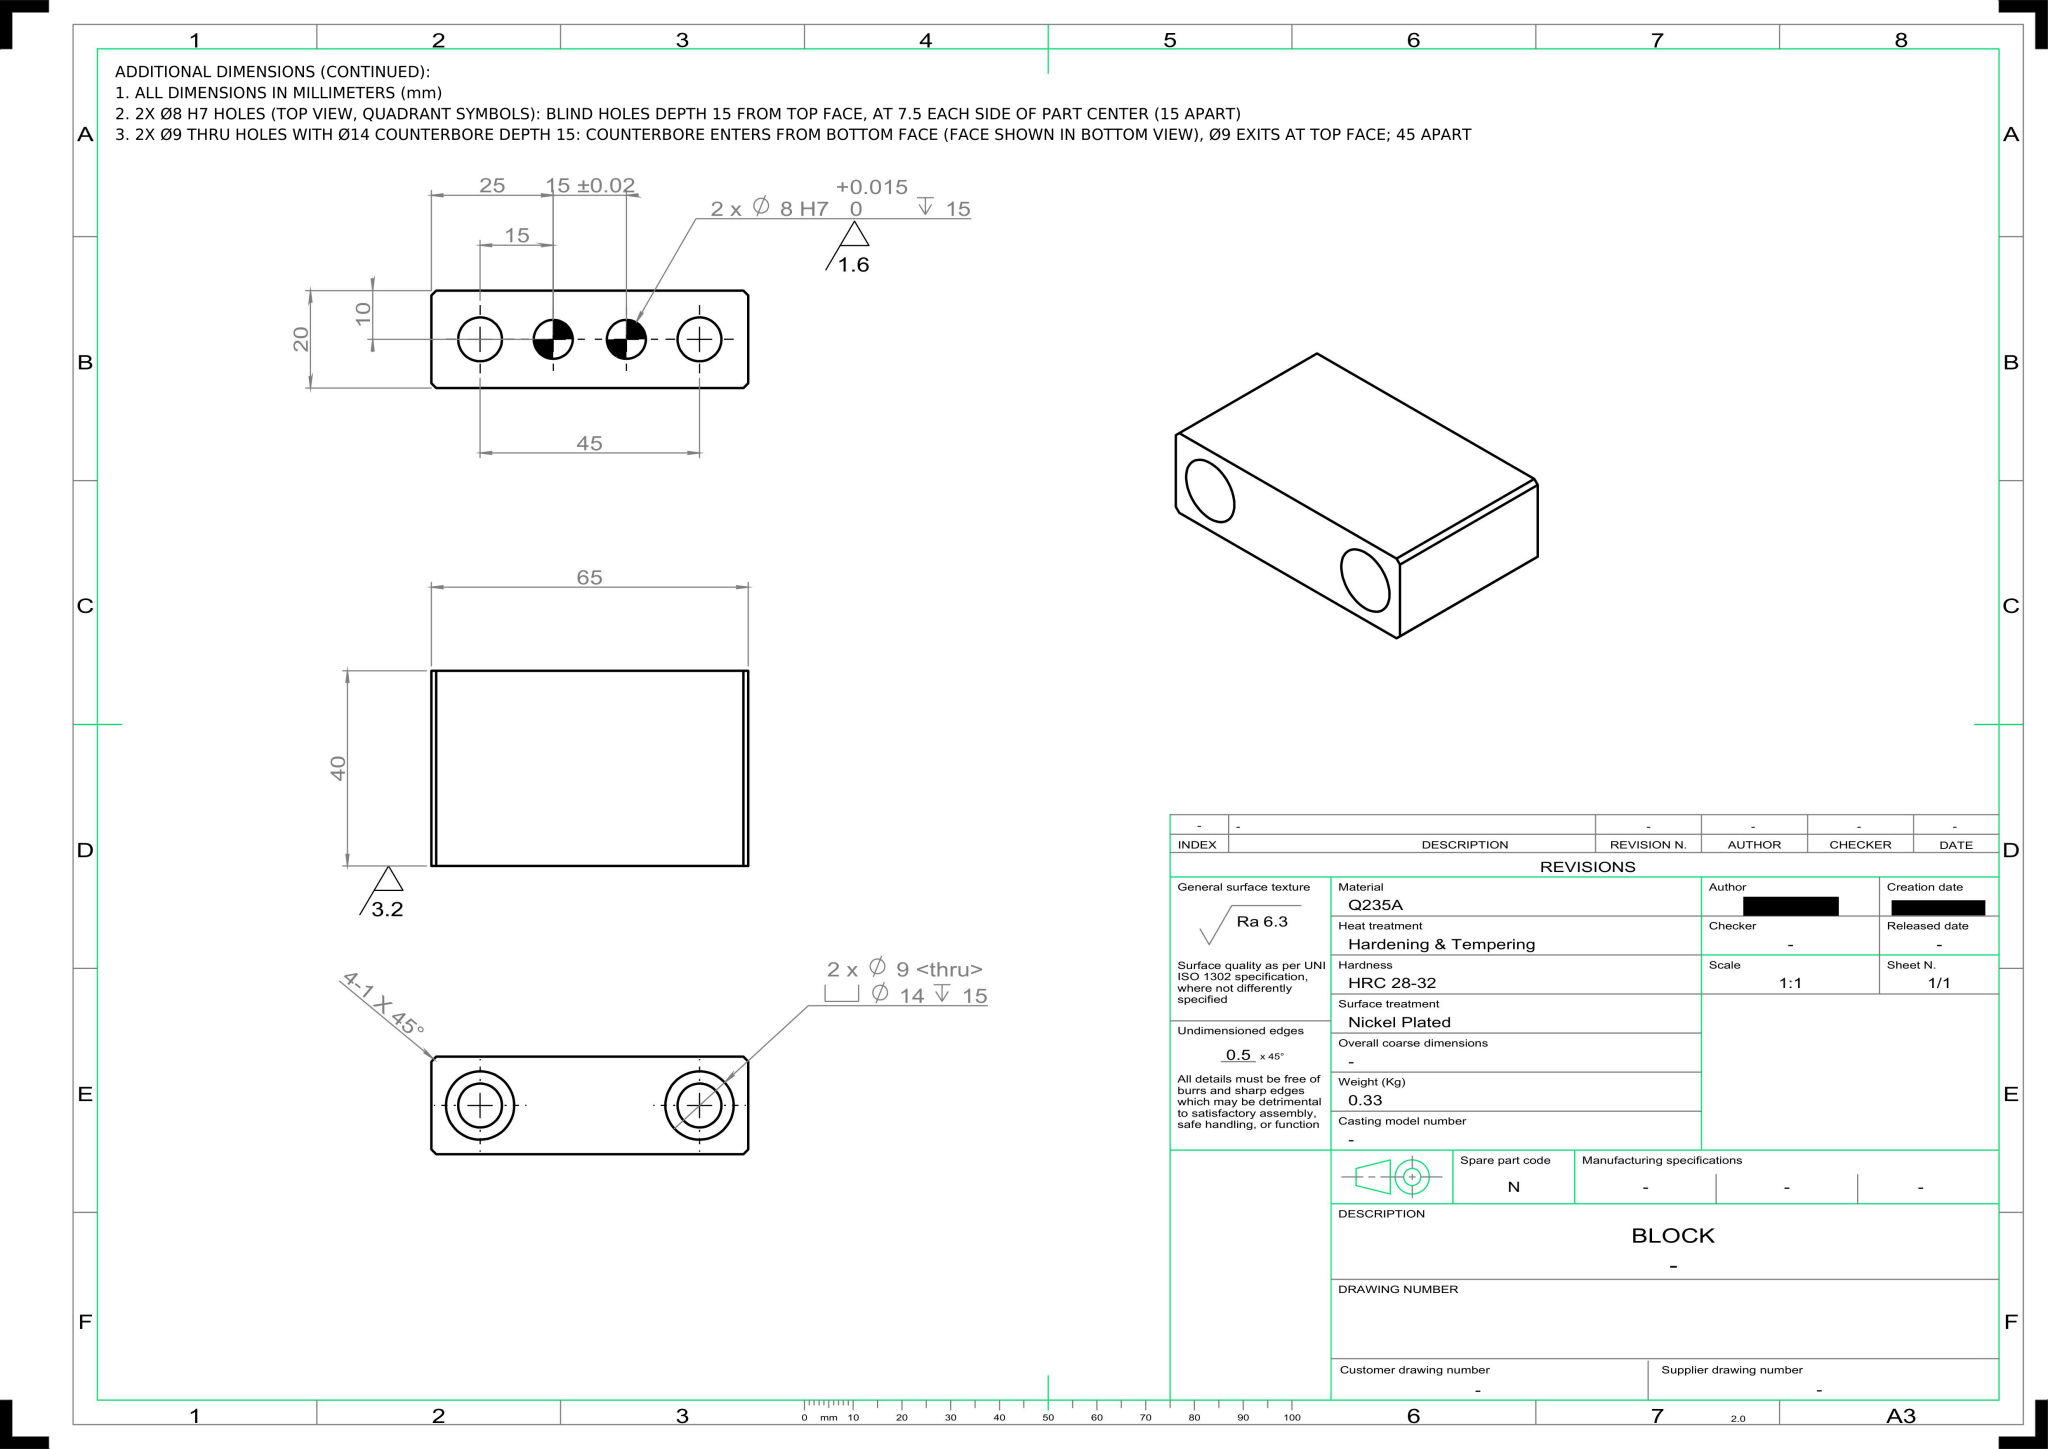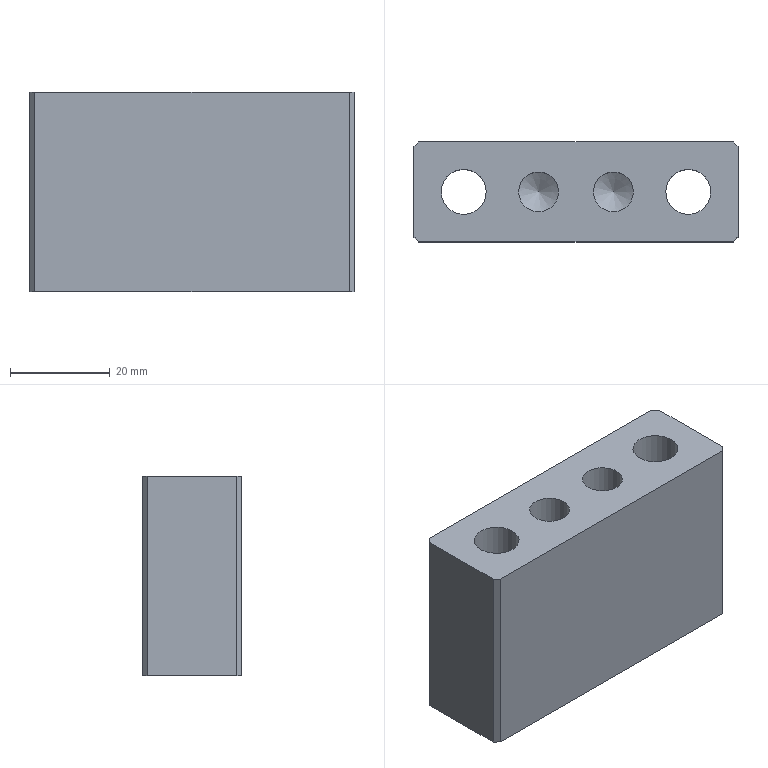Part | NX | mm | 1 solid | 20 faces | box 65 x 20 x 40 mm | volume 42532 mm3 | plane 12 | cylinder 6 | cone 2 | commonest cylinder face diameters 9 x2 14 x2 8 x2
STEP:
#1=CARTESIAN_POINT('',(0.,0.,0.));
#2=DIRECTION('',(0.,0.,1.));
#3=DIRECTION('',(1.,0.,0.));
#4=AXIS2_PLACEMENT_3D('',#1,#2,#3);
#5=(LENGTH_UNIT()NAMED_UNIT(*)SI_UNIT(.MILLI.,.METRE.));
#6=UNCERTAINTY_MEASURE_WITH_UNIT(LENGTH_MEASURE(0.00002),#5,'','');
#7=(NAMED_UNIT(*)PLANE_ANGLE_UNIT()SI_UNIT($,.RADIAN.));
#8=PLANE_ANGLE_MEASURE_WITH_UNIT(PLANE_ANGLE_MEASURE(0.01745),#7);
#9=DIMENSIONAL_EXPONENTS(0.,0.,0.,0.,0.,0.,0.);
#10=(CONVERSION_BASED_UNIT('',#8)NAMED_UNIT(#9)PLANE_ANGLE_UNIT());
#11=(NAMED_UNIT(*)SI_UNIT($,.STERADIAN.)SOLID_ANGLE_UNIT());
#12=(GEOMETRIC_REPRESENTATION_CONTEXT(3)GLOBAL_UNCERTAINTY_ASSIGNED_CONTEXT((#6))GLOBAL_UNIT_ASSIGNED_CONTEXT((#5,#10,#11))REPRESENTATION_CONTEXT('',''));
#13=SHAPE_REPRESENTATION('',(#4),#12);
#14=CARTESIAN_POINT('',(-32.5,9.,0.));
#15=VERTEX_POINT('',#14);
#16=CARTESIAN_POINT('',(-32.5,-9.,0.));
#17=VERTEX_POINT('',#16);
#18=CARTESIAN_POINT('',(-32.5,9.,0.));
#19=DIRECTION('',(0.,-1.,0.));
#20=VECTOR('',#19,1.);
#21=LINE('',#18,#20);
#22=EDGE_CURVE('',#15,#17,#21,.T.);
#23=ORIENTED_EDGE('',*,*,#22,.F.);
#24=CARTESIAN_POINT('',(-32.5,9.,-40.));
#25=VERTEX_POINT('',#24);
#26=CARTESIAN_POINT('',(-32.5,9.,-40.));
#27=DIRECTION('',(0.,0.,1.));
#28=VECTOR('',#27,1.);
#29=LINE('',#26,#28);
#30=EDGE_CURVE('',#25,#15,#29,.T.);
#31=ORIENTED_EDGE('',*,*,#30,.F.);
#32=CARTESIAN_POINT('',(-32.5,-9.,-40.));
#33=VERTEX_POINT('',#32);
#34=CARTESIAN_POINT('',(-32.5,9.,-40.));
#35=DIRECTION('',(0.,-1.,0.));
#36=VECTOR('',#35,1.);
#37=LINE('',#34,#36);
#38=EDGE_CURVE('',#25,#33,#37,.T.);
#39=ORIENTED_EDGE('',*,*,#38,.T.);
#40=CARTESIAN_POINT('',(-32.5,-9.,-40.));
#41=DIRECTION('',(0.,0.,1.));
#42=VECTOR('',#41,1.);
#43=LINE('',#40,#42);
#44=EDGE_CURVE('',#33,#17,#43,.T.);
#45=ORIENTED_EDGE('',*,*,#44,.T.);
#46=EDGE_LOOP('',(#23,#31,#39,#45));
#47=FACE_OUTER_BOUND('',#46,.T.);
#48=CARTESIAN_POINT('',(-32.5,9.,-40.));
#49=DIRECTION('',(-1.,0.,0.));
#50=DIRECTION('',(0.,0.,1.));
#51=AXIS2_PLACEMENT_3D('',#48,#49,#50);
#52=PLANE('',#51);
#53=ADVANCED_FACE('',(#47),#52,.T.);
#54=CARTESIAN_POINT('',(-31.5,-10.,0.));
#55=VERTEX_POINT('',#54);
#56=CARTESIAN_POINT('',(-32.5,-9.,0.));
#57=DIRECTION('',(0.7071,-0.7071,0.));
#58=VECTOR('',#57,1.);
#59=LINE('',#56,#58);
#60=EDGE_CURVE('',#17,#55,#59,.T.);
#61=ORIENTED_EDGE('',*,*,#60,.F.);
#62=ORIENTED_EDGE('',*,*,#44,.F.);
#63=CARTESIAN_POINT('',(-31.5,-10.,-40.));
#64=VERTEX_POINT('',#63);
#65=CARTESIAN_POINT('',(-32.5,-9.,-40.));
#66=DIRECTION('',(0.7071,-0.7071,0.));
#67=VECTOR('',#66,1.);
#68=LINE('',#65,#67);
#69=EDGE_CURVE('',#33,#64,#68,.T.);
#70=ORIENTED_EDGE('',*,*,#69,.T.);
#71=CARTESIAN_POINT('',(-31.5,-10.,-40.));
#72=DIRECTION('',(0.,0.,1.));
#73=VECTOR('',#72,1.);
#74=LINE('',#71,#73);
#75=EDGE_CURVE('',#64,#55,#74,.T.);
#76=ORIENTED_EDGE('',*,*,#75,.T.);
#77=EDGE_LOOP('',(#61,#62,#70,#76));
#78=FACE_OUTER_BOUND('',#77,.T.);
#79=CARTESIAN_POINT('',(-32.5,-9.,-40.));
#80=DIRECTION('',(-0.7071,-0.7071,0.));
#81=DIRECTION('',(0.7071,-0.7071,0.));
#82=AXIS2_PLACEMENT_3D('',#79,#80,#81);
#83=PLANE('',#82);
#84=ADVANCED_FACE('',(#78),#83,.T.);
#85=CARTESIAN_POINT('',(31.5,-10.,0.));
#86=VERTEX_POINT('',#85);
#87=CARTESIAN_POINT('',(-31.5,-10.,0.));
#88=DIRECTION('',(1.,0.,0.));
#89=VECTOR('',#88,1.);
#90=LINE('',#87,#89);
#91=EDGE_CURVE('',#55,#86,#90,.T.);
#92=ORIENTED_EDGE('',*,*,#91,.F.);
#93=ORIENTED_EDGE('',*,*,#75,.F.);
#94=CARTESIAN_POINT('',(31.5,-10.,-40.));
#95=VERTEX_POINT('',#94);
#96=CARTESIAN_POINT('',(-31.5,-10.,-40.));
#97=DIRECTION('',(1.,0.,0.));
#98=VECTOR('',#97,1.);
#99=LINE('',#96,#98);
#100=EDGE_CURVE('',#64,#95,#99,.T.);
#101=ORIENTED_EDGE('',*,*,#100,.T.);
#102=CARTESIAN_POINT('',(31.5,-10.,-40.));
#103=DIRECTION('',(0.,0.,1.));
#104=VECTOR('',#103,1.);
#105=LINE('',#102,#104);
#106=EDGE_CURVE('',#95,#86,#105,.T.);
#107=ORIENTED_EDGE('',*,*,#106,.T.);
#108=EDGE_LOOP('',(#92,#93,#101,#107));
#109=FACE_OUTER_BOUND('',#108,.T.);
#110=CARTESIAN_POINT('',(-31.5,-10.,-40.));
#111=DIRECTION('',(0.,-1.,0.));
#112=DIRECTION('',(0.,0.,-1.));
#113=AXIS2_PLACEMENT_3D('',#110,#111,#112);
#114=PLANE('',#113);
#115=ADVANCED_FACE('',(#109),#114,.T.);
#116=CARTESIAN_POINT('',(32.5,-9.,0.));
#117=VERTEX_POINT('',#116);
#118=CARTESIAN_POINT('',(31.5,-10.,0.));
#119=DIRECTION('',(0.7071,0.7071,0.));
#120=VECTOR('',#119,1.);
#121=LINE('',#118,#120);
#122=EDGE_CURVE('',#86,#117,#121,.T.);
#123=ORIENTED_EDGE('',*,*,#122,.F.);
#124=ORIENTED_EDGE('',*,*,#106,.F.);
#125=CARTESIAN_POINT('',(32.5,-9.,-40.));
#126=VERTEX_POINT('',#125);
#127=CARTESIAN_POINT('',(31.5,-10.,-40.));
#128=DIRECTION('',(0.7071,0.7071,0.));
#129=VECTOR('',#128,1.);
#130=LINE('',#127,#129);
#131=EDGE_CURVE('',#95,#126,#130,.T.);
#132=ORIENTED_EDGE('',*,*,#131,.T.);
#133=CARTESIAN_POINT('',(32.5,-9.,-40.));
#134=DIRECTION('',(0.,0.,1.));
#135=VECTOR('',#134,1.);
#136=LINE('',#133,#135);
#137=EDGE_CURVE('',#126,#117,#136,.T.);
#138=ORIENTED_EDGE('',*,*,#137,.T.);
#139=EDGE_LOOP('',(#123,#124,#132,#138));
#140=FACE_OUTER_BOUND('',#139,.T.);
#141=CARTESIAN_POINT('',(31.5,-10.,-40.));
#142=DIRECTION('',(0.7071,-0.7071,0.));
#143=DIRECTION('',(0.7071,0.7071,0.));
#144=AXIS2_PLACEMENT_3D('',#141,#142,#143);
#145=PLANE('',#144);
#146=ADVANCED_FACE('',(#140),#145,.T.);
#147=CARTESIAN_POINT('',(32.5,9.,0.));
#148=VERTEX_POINT('',#147);
#149=CARTESIAN_POINT('',(32.5,-9.,0.));
#150=DIRECTION('',(0.,1.,0.));
#151=VECTOR('',#150,1.);
#152=LINE('',#149,#151);
#153=EDGE_CURVE('',#117,#148,#152,.T.);
#154=ORIENTED_EDGE('',*,*,#153,.F.);
#155=ORIENTED_EDGE('',*,*,#137,.F.);
#156=CARTESIAN_POINT('',(32.5,9.,-40.));
#157=VERTEX_POINT('',#156);
#158=CARTESIAN_POINT('',(32.5,-9.,-40.));
#159=DIRECTION('',(0.,1.,0.));
#160=VECTOR('',#159,1.);
#161=LINE('',#158,#160);
#162=EDGE_CURVE('',#126,#157,#161,.T.);
#163=ORIENTED_EDGE('',*,*,#162,.T.);
#164=CARTESIAN_POINT('',(32.5,9.,-40.));
#165=DIRECTION('',(0.,0.,1.));
#166=VECTOR('',#165,1.);
#167=LINE('',#164,#166);
#168=EDGE_CURVE('',#157,#148,#167,.T.);
#169=ORIENTED_EDGE('',*,*,#168,.T.);
#170=EDGE_LOOP('',(#154,#155,#163,#169));
#171=FACE_OUTER_BOUND('',#170,.T.);
#172=CARTESIAN_POINT('',(32.5,-9.,-40.));
#173=DIRECTION('',(1.,0.,0.));
#174=DIRECTION('',(0.,0.,-1.));
#175=AXIS2_PLACEMENT_3D('',#172,#173,#174);
#176=PLANE('',#175);
#177=ADVANCED_FACE('',(#171),#176,.T.);
#178=CARTESIAN_POINT('',(31.5,10.,0.));
#179=VERTEX_POINT('',#178);
#180=CARTESIAN_POINT('',(32.5,9.,0.));
#181=DIRECTION('',(-0.7071,0.7071,0.));
#182=VECTOR('',#181,1.);
#183=LINE('',#180,#182);
#184=EDGE_CURVE('',#148,#179,#183,.T.);
#185=ORIENTED_EDGE('',*,*,#184,.F.);
#186=ORIENTED_EDGE('',*,*,#168,.F.);
#187=CARTESIAN_POINT('',(31.5,10.,-40.));
#188=VERTEX_POINT('',#187);
#189=CARTESIAN_POINT('',(32.5,9.,-40.));
#190=DIRECTION('',(-0.7071,0.7071,0.));
#191=VECTOR('',#190,1.);
#192=LINE('',#189,#191);
#193=EDGE_CURVE('',#157,#188,#192,.T.);
#194=ORIENTED_EDGE('',*,*,#193,.T.);
#195=CARTESIAN_POINT('',(31.5,10.,-40.));
#196=DIRECTION('',(0.,0.,1.));
#197=VECTOR('',#196,1.);
#198=LINE('',#195,#197);
#199=EDGE_CURVE('',#188,#179,#198,.T.);
#200=ORIENTED_EDGE('',*,*,#199,.T.);
#201=EDGE_LOOP('',(#185,#186,#194,#200));
#202=FACE_OUTER_BOUND('',#201,.T.);
#203=CARTESIAN_POINT('',(32.5,9.,-40.));
#204=DIRECTION('',(0.7071,0.7071,0.));
#205=DIRECTION('',(-0.7071,0.7071,0.));
#206=AXIS2_PLACEMENT_3D('',#203,#204,#205);
#207=PLANE('',#206);
#208=ADVANCED_FACE('',(#202),#207,.T.);
#209=CARTESIAN_POINT('',(-31.5,10.,0.));
#210=VERTEX_POINT('',#209);
#211=CARTESIAN_POINT('',(31.5,10.,0.));
#212=DIRECTION('',(-1.,0.,0.));
#213=VECTOR('',#212,1.);
#214=LINE('',#211,#213);
#215=EDGE_CURVE('',#179,#210,#214,.T.);
#216=ORIENTED_EDGE('',*,*,#215,.F.);
#217=ORIENTED_EDGE('',*,*,#199,.F.);
#218=CARTESIAN_POINT('',(-31.5,10.,-40.));
#219=VERTEX_POINT('',#218);
#220=CARTESIAN_POINT('',(31.5,10.,-40.));
#221=DIRECTION('',(-1.,0.,0.));
#222=VECTOR('',#221,1.);
#223=LINE('',#220,#222);
#224=EDGE_CURVE('',#188,#219,#223,.T.);
#225=ORIENTED_EDGE('',*,*,#224,.T.);
#226=CARTESIAN_POINT('',(-31.5,10.,-40.));
#227=DIRECTION('',(0.,0.,1.));
#228=VECTOR('',#227,1.);
#229=LINE('',#226,#228);
#230=EDGE_CURVE('',#219,#210,#229,.T.);
#231=ORIENTED_EDGE('',*,*,#230,.T.);
#232=EDGE_LOOP('',(#216,#217,#225,#231));
#233=FACE_OUTER_BOUND('',#232,.T.);
#234=CARTESIAN_POINT('',(31.5,10.,-40.));
#235=DIRECTION('',(0.,1.,0.));
#236=DIRECTION('',(0.,0.,1.));
#237=AXIS2_PLACEMENT_3D('',#234,#235,#236);
#238=PLANE('',#237);
#239=ADVANCED_FACE('',(#233),#238,.T.);
#240=CARTESIAN_POINT('',(-31.5,10.,0.));
#241=DIRECTION('',(-0.7071,-0.7071,0.));
#242=VECTOR('',#241,1.);
#243=LINE('',#240,#242);
#244=EDGE_CURVE('',#210,#15,#243,.T.);
#245=ORIENTED_EDGE('',*,*,#244,.F.);
#246=ORIENTED_EDGE('',*,*,#230,.F.);
#247=CARTESIAN_POINT('',(-31.5,10.,-40.));
#248=DIRECTION('',(-0.7071,-0.7071,0.));
#249=VECTOR('',#248,1.);
#250=LINE('',#247,#249);
#251=EDGE_CURVE('',#219,#25,#250,.T.);
#252=ORIENTED_EDGE('',*,*,#251,.T.);
#253=ORIENTED_EDGE('',*,*,#30,.T.);
#254=EDGE_LOOP('',(#245,#246,#252,#253));
#255=FACE_OUTER_BOUND('',#254,.T.);
#256=CARTESIAN_POINT('',(-31.5,10.,-40.));
#257=DIRECTION('',(-0.7071,0.7071,0.));
#258=DIRECTION('',(-0.7071,-0.7071,0.));
#259=AXIS2_PLACEMENT_3D('',#256,#257,#258);
#260=PLANE('',#259);
#261=ADVANCED_FACE('',(#255),#260,.T.);
#262=CARTESIAN_POINT('',(29.5,-0.,-40.));
#263=VERTEX_POINT('',#262);
#264=CARTESIAN_POINT('',(22.5,-0.,-40.));
#265=DIRECTION('',(0.,0.,1.));
#266=DIRECTION('',(1.,0.,0.));
#267=AXIS2_PLACEMENT_3D('',#264,#265,#266);
#268=CIRCLE('',#267,7.);
#269=EDGE_CURVE('',#263,#263,#268,.T.);
#270=ORIENTED_EDGE('',*,*,#269,.T.);
#271=EDGE_LOOP('',(#270));
#272=FACE_BOUND('',#271,.T.);
#273=CARTESIAN_POINT('',(-15.5,-0.,-40.));
#274=VERTEX_POINT('',#273);
#275=CARTESIAN_POINT('',(-22.5,-0.,-40.));
#276=DIRECTION('',(0.,0.,1.));
#277=DIRECTION('',(1.,0.,0.));
#278=AXIS2_PLACEMENT_3D('',#275,#276,#277);
#279=CIRCLE('',#278,7.);
#280=EDGE_CURVE('',#274,#274,#279,.T.);
#281=ORIENTED_EDGE('',*,*,#280,.T.);
#282=EDGE_LOOP('',(#281));
#283=FACE_BOUND('',#282,.T.);
#284=ORIENTED_EDGE('',*,*,#38,.F.);
#285=ORIENTED_EDGE('',*,*,#251,.F.);
#286=ORIENTED_EDGE('',*,*,#224,.F.);
#287=ORIENTED_EDGE('',*,*,#193,.F.);
#288=ORIENTED_EDGE('',*,*,#162,.F.);
#289=ORIENTED_EDGE('',*,*,#131,.F.);
#290=ORIENTED_EDGE('',*,*,#100,.F.);
#291=ORIENTED_EDGE('',*,*,#69,.F.);
#292=EDGE_LOOP('',(#284,#285,#286,#287,#288,#289,#290,#291));
#293=FACE_BOUND('',#292,.T.);
#294=CARTESIAN_POINT('',(0.,0.,-40.));
#295=DIRECTION('',(0.,0.,1.));
#296=DIRECTION('',(1.,0.,0.));
#297=AXIS2_PLACEMENT_3D('',#294,#295,#296);
#298=PLANE('',#297);
#299=ADVANCED_FACE('',(#272,#283,#293),#298,.F.);
#300=CARTESIAN_POINT('',(3.5,0.,0.));
#301=VERTEX_POINT('',#300);
#302=CARTESIAN_POINT('',(7.5,0.,0.));
#303=DIRECTION('',(0.,0.,-1.));
#304=DIRECTION('',(-1.,0.,0.));
#305=AXIS2_PLACEMENT_3D('',#302,#303,#304);
#306=CIRCLE('',#305,4.);
#307=EDGE_CURVE('',#301,#301,#306,.T.);
#308=ORIENTED_EDGE('',*,*,#307,.T.);
#309=EDGE_LOOP('',(#308));
#310=FACE_BOUND('',#309,.T.);
#311=CARTESIAN_POINT('',(-11.5,0.,0.));
#312=VERTEX_POINT('',#311);
#313=CARTESIAN_POINT('',(-7.5,0.,0.));
#314=DIRECTION('',(0.,0.,-1.));
#315=DIRECTION('',(-1.,0.,0.));
#316=AXIS2_PLACEMENT_3D('',#313,#314,#315);
#317=CIRCLE('',#316,4.);
#318=EDGE_CURVE('',#312,#312,#317,.T.);
#319=ORIENTED_EDGE('',*,*,#318,.T.);
#320=EDGE_LOOP('',(#319));
#321=FACE_BOUND('',#320,.T.);
#322=CARTESIAN_POINT('',(27.,-0.,0.));
#323=VERTEX_POINT('',#322);
#324=CARTESIAN_POINT('',(22.5,-0.,0.));
#325=DIRECTION('',(0.,0.,1.));
#326=DIRECTION('',(1.,0.,0.));
#327=AXIS2_PLACEMENT_3D('',#324,#325,#326);
#328=CIRCLE('',#327,4.5);
#329=EDGE_CURVE('',#323,#323,#328,.T.);
#330=ORIENTED_EDGE('',*,*,#329,.F.);
#331=EDGE_LOOP('',(#330));
#332=FACE_BOUND('',#331,.T.);
#333=CARTESIAN_POINT('',(-18.,-0.,0.));
#334=VERTEX_POINT('',#333);
#335=CARTESIAN_POINT('',(-22.5,-0.,0.));
#336=DIRECTION('',(0.,0.,1.));
#337=DIRECTION('',(1.,0.,0.));
#338=AXIS2_PLACEMENT_3D('',#335,#336,#337);
#339=CIRCLE('',#338,4.5);
#340=EDGE_CURVE('',#334,#334,#339,.T.);
#341=ORIENTED_EDGE('',*,*,#340,.F.);
#342=EDGE_LOOP('',(#341));
#343=FACE_BOUND('',#342,.T.);
#344=ORIENTED_EDGE('',*,*,#22,.T.);
#345=ORIENTED_EDGE('',*,*,#60,.T.);
#346=ORIENTED_EDGE('',*,*,#91,.T.);
#347=ORIENTED_EDGE('',*,*,#122,.T.);
#348=ORIENTED_EDGE('',*,*,#153,.T.);
#349=ORIENTED_EDGE('',*,*,#184,.T.);
#350=ORIENTED_EDGE('',*,*,#215,.T.);
#351=ORIENTED_EDGE('',*,*,#244,.T.);
#352=EDGE_LOOP('',(#344,#345,#346,#347,#348,#349,#350,#351));
#353=FACE_BOUND('',#352,.T.);
#354=CARTESIAN_POINT('',(0.,0.,0.));
#355=DIRECTION('',(0.,0.,1.));
#356=DIRECTION('',(1.,0.,0.));
#357=AXIS2_PLACEMENT_3D('',#354,#355,#356);
#358=PLANE('',#357);
#359=ADVANCED_FACE('',(#310,#321,#332,#343,#353),#358,.T.);
#360=ORIENTED_EDGE('',*,*,#340,.T.);
#361=EDGE_LOOP('',(#360));
#362=FACE_BOUND('',#361,.T.);
#363=CARTESIAN_POINT('',(-18.,-0.,-25.));
#364=VERTEX_POINT('',#363);
#365=CARTESIAN_POINT('',(-22.5,-0.,-25.));
#366=DIRECTION('',(0.,0.,-1.));
#367=DIRECTION('',(1.,0.,0.));
#368=AXIS2_PLACEMENT_3D('',#365,#366,#367);
#369=CIRCLE('',#368,4.5);
#370=EDGE_CURVE('',#364,#364,#369,.T.);
#371=ORIENTED_EDGE('',*,*,#370,.T.);
#372=EDGE_LOOP('',(#371));
#373=FACE_BOUND('',#372,.T.);
#374=CARTESIAN_POINT('',(-22.5,-0.,17.105));
#375=DIRECTION('',(0.,0.,1.));
#376=DIRECTION('',(1.,0.,0.));
#377=AXIS2_PLACEMENT_3D('',#374,#375,#376);
#378=CYLINDRICAL_SURFACE('',#377,4.5);
#379=ADVANCED_FACE('',(#362,#373),#378,.F.);
#380=ORIENTED_EDGE('',*,*,#370,.F.);
#381=EDGE_LOOP('',(#380));
#382=FACE_BOUND('',#381,.T.);
#383=CARTESIAN_POINT('',(-15.5,-0.,-25.));
#384=VERTEX_POINT('',#383);
#385=CARTESIAN_POINT('',(-22.5,-0.,-25.));
#386=DIRECTION('',(0.,0.,-1.));
#387=DIRECTION('',(1.,0.,0.));
#388=AXIS2_PLACEMENT_3D('',#385,#386,#387);
#389=CIRCLE('',#388,7.);
#390=EDGE_CURVE('',#384,#384,#389,.T.);
#391=ORIENTED_EDGE('',*,*,#390,.T.);
#392=EDGE_LOOP('',(#391));
#393=FACE_BOUND('',#392,.T.);
#394=CARTESIAN_POINT('',(-22.5,-0.,-25.));
#395=DIRECTION('',(0.,0.,1.));
#396=DIRECTION('',(1.,0.,0.));
#397=AXIS2_PLACEMENT_3D('',#394,#395,#396);
#398=PLANE('',#397);
#399=ADVANCED_FACE('',(#382,#393),#398,.F.);
#400=ORIENTED_EDGE('',*,*,#390,.F.);
#401=EDGE_LOOP('',(#400));
#402=FACE_BOUND('',#401,.T.);
#403=ORIENTED_EDGE('',*,*,#280,.F.);
#404=EDGE_LOOP('',(#403));
#405=FACE_BOUND('',#404,.T.);
#406=CARTESIAN_POINT('',(-22.5,-0.,-40.));
#407=DIRECTION('',(0.,0.,1.));
#408=DIRECTION('',(1.,0.,0.));
#409=AXIS2_PLACEMENT_3D('',#406,#407,#408);
#410=CYLINDRICAL_SURFACE('',#409,7.);
#411=ADVANCED_FACE('',(#402,#405),#410,.F.);
#412=ORIENTED_EDGE('',*,*,#329,.T.);
#413=EDGE_LOOP('',(#412));
#414=FACE_BOUND('',#413,.T.);
#415=CARTESIAN_POINT('',(27.,-0.,-25.));
#416=VERTEX_POINT('',#415);
#417=CARTESIAN_POINT('',(22.5,-0.,-25.));
#418=DIRECTION('',(0.,0.,-1.));
#419=DIRECTION('',(1.,0.,0.));
#420=AXIS2_PLACEMENT_3D('',#417,#418,#419);
#421=CIRCLE('',#420,4.5);
#422=EDGE_CURVE('',#416,#416,#421,.T.);
#423=ORIENTED_EDGE('',*,*,#422,.T.);
#424=EDGE_LOOP('',(#423));
#425=FACE_BOUND('',#424,.T.);
#426=CARTESIAN_POINT('',(22.5,-0.,17.105));
#427=DIRECTION('',(0.,0.,1.));
#428=DIRECTION('',(1.,0.,0.));
#429=AXIS2_PLACEMENT_3D('',#426,#427,#428);
#430=CYLINDRICAL_SURFACE('',#429,4.5);
#431=ADVANCED_FACE('',(#414,#425),#430,.F.);
#432=ORIENTED_EDGE('',*,*,#422,.F.);
#433=EDGE_LOOP('',(#432));
#434=FACE_BOUND('',#433,.T.);
#435=CARTESIAN_POINT('',(29.5,-0.,-25.));
#436=VERTEX_POINT('',#435);
#437=CARTESIAN_POINT('',(22.5,-0.,-25.));
#438=DIRECTION('',(0.,0.,-1.));
#439=DIRECTION('',(1.,0.,0.));
#440=AXIS2_PLACEMENT_3D('',#437,#438,#439);
#441=CIRCLE('',#440,7.);
#442=EDGE_CURVE('',#436,#436,#441,.T.);
#443=ORIENTED_EDGE('',*,*,#442,.T.);
#444=EDGE_LOOP('',(#443));
#445=FACE_BOUND('',#444,.T.);
#446=CARTESIAN_POINT('',(22.5,-0.,-25.));
#447=DIRECTION('',(0.,0.,1.));
#448=DIRECTION('',(1.,0.,0.));
#449=AXIS2_PLACEMENT_3D('',#446,#447,#448);
#450=PLANE('',#449);
#451=ADVANCED_FACE('',(#434,#445),#450,.F.);
#452=ORIENTED_EDGE('',*,*,#442,.F.);
#453=EDGE_LOOP('',(#452));
#454=FACE_BOUND('',#453,.T.);
#455=ORIENTED_EDGE('',*,*,#269,.F.);
#456=EDGE_LOOP('',(#455));
#457=FACE_BOUND('',#456,.T.);
#458=CARTESIAN_POINT('',(22.5,-0.,-40.));
#459=DIRECTION('',(0.,0.,1.));
#460=DIRECTION('',(1.,0.,0.));
#461=AXIS2_PLACEMENT_3D('',#458,#459,#460);
#462=CYLINDRICAL_SURFACE('',#461,7.);
#463=ADVANCED_FACE('',(#454,#457),#462,.F.);
#464=CARTESIAN_POINT('',(-11.5,0.,-15.));
#465=VERTEX_POINT('',#464);
#466=CARTESIAN_POINT('',(-7.5,0.,-15.));
#467=DIRECTION('',(0.,0.,1.));
#468=DIRECTION('',(-1.,0.,0.));
#469=AXIS2_PLACEMENT_3D('',#466,#467,#468);
#470=CIRCLE('',#469,4.);
#471=EDGE_CURVE('',#465,#465,#470,.T.);
#472=ORIENTED_EDGE('',*,*,#471,.T.);
#473=EDGE_LOOP('',(#472));
#474=FACE_BOUND('',#473,.T.);
#475=CARTESIAN_POINT('',(-7.5,0.,-17.403));
#476=VERTEX_POINT('',#475);
#477=VERTEX_LOOP('',#476);
#478=FACE_BOUND('',#477,.T.);
#479=CARTESIAN_POINT('',(-7.5,0.,-15.));
#480=DIRECTION('',(0.,0.,1.));
#481=DIRECTION('',(1.,0.,-0.));
#482=AXIS2_PLACEMENT_3D('',#479,#480,#481);
#483=CONICAL_SURFACE('',#482,4.,59.);
#484=ADVANCED_FACE('',(#474,#478),#483,.F.);
#485=ORIENTED_EDGE('',*,*,#471,.F.);
#486=EDGE_LOOP('',(#485));
#487=FACE_BOUND('',#486,.T.);
#488=ORIENTED_EDGE('',*,*,#318,.F.);
#489=EDGE_LOOP('',(#488));
#490=FACE_BOUND('',#489,.T.);
#491=CARTESIAN_POINT('',(-7.5,0.,0.));
#492=DIRECTION('',(0.,0.,-1.));
#493=DIRECTION('',(-1.,0.,0.));
#494=AXIS2_PLACEMENT_3D('',#491,#492,#493);
#495=CYLINDRICAL_SURFACE('',#494,4.);
#496=ADVANCED_FACE('',(#487,#490),#495,.F.);
#497=CARTESIAN_POINT('',(3.5,0.,-15.));
#498=VERTEX_POINT('',#497);
#499=CARTESIAN_POINT('',(7.5,0.,-15.));
#500=DIRECTION('',(0.,0.,1.));
#501=DIRECTION('',(-1.,0.,0.));
#502=AXIS2_PLACEMENT_3D('',#499,#500,#501);
#503=CIRCLE('',#502,4.);
#504=EDGE_CURVE('',#498,#498,#503,.T.);
#505=ORIENTED_EDGE('',*,*,#504,.T.);
#506=EDGE_LOOP('',(#505));
#507=FACE_BOUND('',#506,.T.);
#508=CARTESIAN_POINT('',(7.5,0.,-17.403));
#509=VERTEX_POINT('',#508);
#510=VERTEX_LOOP('',#509);
#511=FACE_BOUND('',#510,.T.);
#512=CARTESIAN_POINT('',(7.5,0.,-15.));
#513=DIRECTION('',(0.,0.,1.));
#514=DIRECTION('',(1.,0.,-0.));
#515=AXIS2_PLACEMENT_3D('',#512,#513,#514);
#516=CONICAL_SURFACE('',#515,4.,59.);
#517=ADVANCED_FACE('',(#507,#511),#516,.F.);
#518=ORIENTED_EDGE('',*,*,#504,.F.);
#519=EDGE_LOOP('',(#518));
#520=FACE_BOUND('',#519,.T.);
#521=ORIENTED_EDGE('',*,*,#307,.F.);
#522=EDGE_LOOP('',(#521));
#523=FACE_BOUND('',#522,.T.);
#524=CARTESIAN_POINT('',(7.5,0.,0.));
#525=DIRECTION('',(0.,0.,-1.));
#526=DIRECTION('',(-1.,0.,0.));
#527=AXIS2_PLACEMENT_3D('',#524,#525,#526);
#528=CYLINDRICAL_SURFACE('',#527,4.);
#529=ADVANCED_FACE('',(#520,#523),#528,.F.);
#530=CLOSED_SHELL('',(#53,#84,#115,#146,#177,#208,#239,#261,#299,#359,#379,#399,#411,#431,#451,#463,#484,#496,#517,#529));
#531=MANIFOLD_SOLID_BREP('',#530);
#532=ADVANCED_BREP_SHAPE_REPRESENTATION('',(#531),#12);
#533=SHAPE_REPRESENTATION_RELATIONSHIP('','',#13,#532);
#534=PRESENTATION_LAYER_ASSIGNMENT('','',(#531));
#535=COLOUR_RGB('',0.4,0.8,1.);
#536=FILL_AREA_STYLE_COLOUR('',#535);
#537=FILL_AREA_STYLE('',(#536));
#538=SURFACE_STYLE_FILL_AREA(#537);
#539=SURFACE_SIDE_STYLE('',(#538));
#540=SURFACE_STYLE_USAGE(.BOTH.,#539);
#541=PRESENTATION_STYLE_ASSIGNMENT((#540));
#542=STYLED_ITEM('',(#541),#531);
#543=MECHANICAL_DESIGN_GEOMETRIC_PRESENTATION_REPRESENTATION('',(#542),#12);